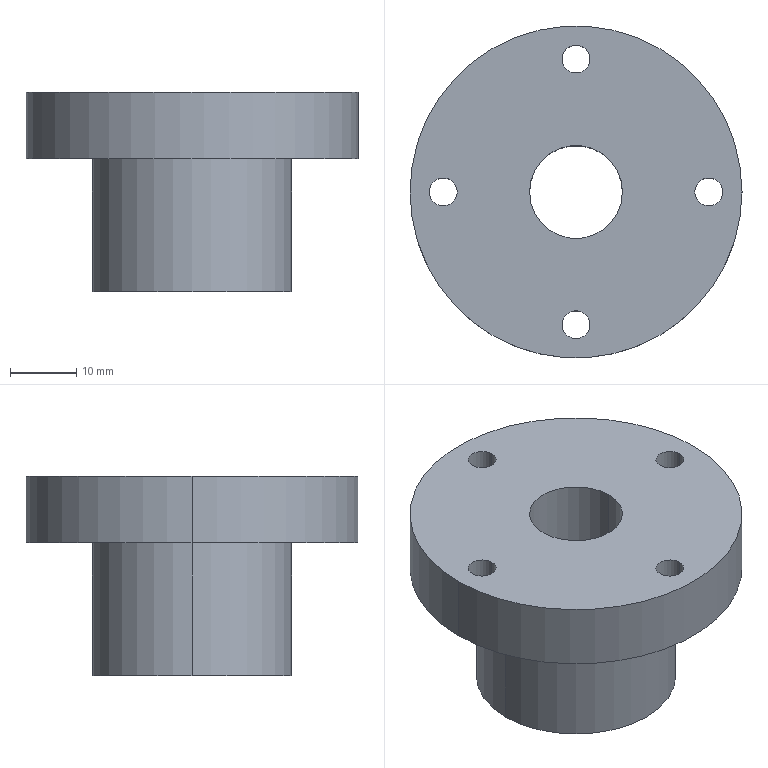Component | SolidWorks | DC-46-018-1 | 1 solid | 17 faces | box 50 x 50 x 30 mm | volume 28600 mm3 | cylinder 14 | plane 3 | commonest cylinder face diameters 4.2 x8 14 x2 30 x2 50 x2
build123d program:
from build123d import *

# Parameters (mm, degrees)
SKETCH1_2_R            = 25
BOSS_EXTRUDE1_DEPTH    = 10
SKETCH2_R              = 15
BOSS_EXTRUDE2_DEPTH    = 20
M14X1_5_TAPPED_HOLE1_D = 12.5
M5_TAPPED_HOLE1_D      = 4.2
SKETCH1_R              = 7
CUT_EXTRUDE1_DEPTH     = 47.368


with BuildPart() as part:
    # Sketch1_2 → Boss-Extrude1 (new body)
    with BuildSketch(Plane.XY):
        Circle(SKETCH1_2_R)
    extrude(amount=BOSS_EXTRUDE1_DEPTH)

    # Sketch2 → Boss-Extrude2 (add)
    with BuildSketch(Plane.XY.offset(10)):
        Circle(SKETCH2_R)
    extrude(amount=BOSS_EXTRUDE2_DEPTH)

    # M14x1.5 Tapped Hole1 (through all)
    with Locations(Plane.XY.offset(30)):
        with Locations((0, 0)):
            Hole(M14X1_5_TAPPED_HOLE1_D / 2)

    # M5 Tapped Hole1 (through all)
    with Locations(Plane.XY.offset(10)):
        with Locations((0, -20), (-20, 0), (0, 20), (20, 0)):
            Hole(M5_TAPPED_HOLE1_D / 2)

    # Sketch1 → Cut-Extrude1 (cut, through all)
    with BuildSketch(Plane(origin=(0, 0, 0), x_dir=(-1, 0, 0), z_dir=(0, 0, -1))):
        Circle(SKETCH1_R)
    extrude(amount=-CUT_EXTRUDE1_DEPTH, mode=Mode.SUBTRACT)


solid = part.part

# Placed as in the assembly
solid = solid.moved(Location((311.865, 195.227, 2075.633), (180, 0, 0)))